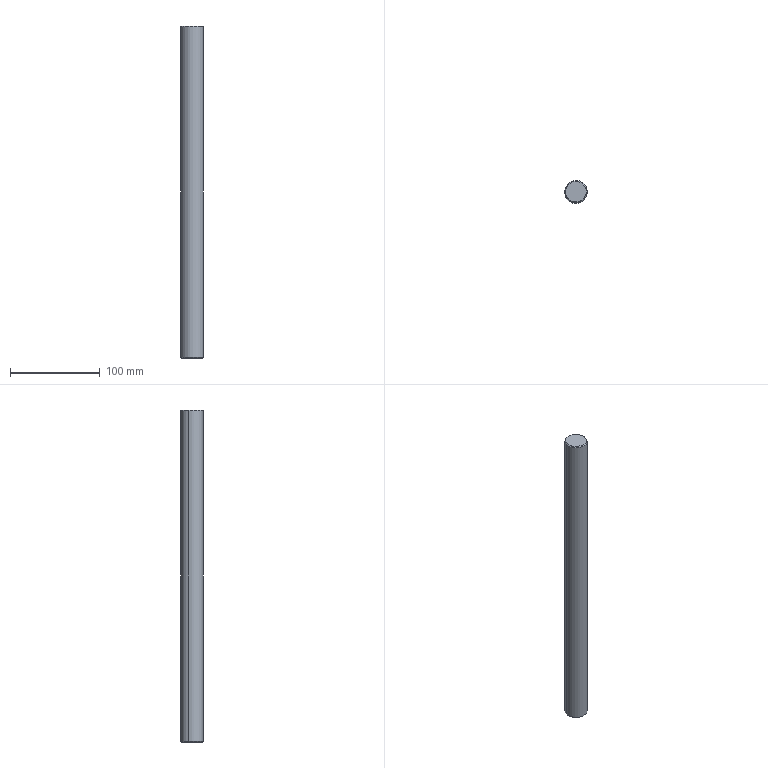Component | SolidWorks | DirectPressureVerticalSeal-1_VerticalSealGuideAxis-2 | 1 solid | 8 faces | box 25 x 25 x 370 mm | volume 181547 mm3 | cone 4 | cylinder 2 | plane 2 | commonest cylinder face diameters 25 x2
build123d program:
from build123d import *


with BuildPart() as part:
    # Sketch1 → Revolve1 (revolve)
    with BuildSketch(Plane.XZ, mode=Mode.PRIVATE) as revolve1_sk:
        Polygon((11.5, 185), (0, 185), (0, -185), (11.5, -185), (12.5, -184), (12.5, 184), align=None)
    revolve(revolve1_sk.sketch.rotate(Axis((0, 0, 185), (0, 0, -1)), 180), axis=Axis((0, 0, 185), (0, 0, -1)))


solid = part.part

# Placed as in the assembly
solid = solid.moved(Location((-98.746, 246.873, 168.5), (0, 0, 0)))
STEP:
#1=COLOUR_RGB('',0.7922,0.8196,0.9333);
#2=FILL_AREA_STYLE_COLOUR('',#1);
#3=FILL_AREA_STYLE('',(#2));
#4=SURFACE_STYLE_FILL_AREA(#3);
#5=SURFACE_SIDE_STYLE('',(#4));
#6=SURFACE_STYLE_USAGE(.BOTH.,#5);
#7=PRESENTATION_STYLE_ASSIGNMENT((#6));
#8=CARTESIAN_POINT('',(-4.323,9.842,-0.6496));
#9=VERTEX_POINT('',#8);
#10=CARTESIAN_POINT('',(-3.452,9.597,-0.6496));
#11=VERTEX_POINT('',#10);
#12=CARTESIAN_POINT('',(-3.888,9.719,-0.6496));
#13=DIRECTION('',(0.,0.,-1.));
#14=DIRECTION('',(-0.9626,0.2708,0.));
#15=AXIS2_PLACEMENT_3D('',#12,#13,#14);
#16=CIRCLE('',#15,0.4528);
#17=EDGE_CURVE('',#9,#11,#16,.T.);
#18=ORIENTED_EDGE('',*,*,#17,.F.);
#19=CARTESIAN_POINT('',(-4.361,9.853,-0.6102));
#20=VERTEX_POINT('',#19);
#21=CARTESIAN_POINT('',(-4.323,9.842,-0.6496));
#22=DIRECTION('',(-0.6807,0.1915,0.7071));
#23=VECTOR('',#22,39.37);
#24=LINE('',#21,#23);
#25=EDGE_CURVE('',#9,#20,#24,.T.);
#26=ORIENTED_EDGE('',*,*,#25,.T.);
#27=CARTESIAN_POINT('',(-3.414,9.586,-0.6102));
#28=VERTEX_POINT('',#27);
#29=CARTESIAN_POINT('',(-3.888,9.719,-0.6102));
#30=DIRECTION('',(0.,0.,-1.));
#31=DIRECTION('',(-0.9626,0.2708,-0.));
#32=AXIS2_PLACEMENT_3D('',#29,#30,#31);
#33=CIRCLE('',#32,0.4921);
#34=EDGE_CURVE('',#20,#28,#33,.T.);
#35=ORIENTED_EDGE('',*,*,#34,.T.);
#36=CARTESIAN_POINT('',(-3.452,9.597,-0.6496));
#37=DIRECTION('',(0.6807,-0.1915,0.7071));
#38=VECTOR('',#37,39.37);
#39=LINE('',#36,#38);
#40=EDGE_CURVE('',#11,#28,#39,.T.);
#41=ORIENTED_EDGE('',*,*,#40,.F.);
#42=EDGE_LOOP('',(#18,#26,#35,#41));
#43=FACE_OUTER_BOUND('',#42,.T.);
#44=CARTESIAN_POINT('',(-3.888,9.719,-0.6496));
#45=DIRECTION('',(-0.,-0.,1.));
#46=DIRECTION('',(0.9626,-0.2708,0.));
#47=AXIS2_PLACEMENT_3D('',#44,#45,#46);
#48=CONICAL_SURFACE('',#47,0.4528,0.7854);
#49=ADVANCED_FACE('',(#43),#48,.T.);
#50=CARTESIAN_POINT('',(-4.361,9.853,13.878));
#51=VERTEX_POINT('',#50);
#52=CARTESIAN_POINT('',(-3.414,9.586,13.878));
#53=VERTEX_POINT('',#52);
#54=CARTESIAN_POINT('',(-3.888,9.719,13.878));
#55=DIRECTION('',(0.,0.,-1.));
#56=DIRECTION('',(-0.9626,0.2708,0.));
#57=AXIS2_PLACEMENT_3D('',#54,#55,#56);
#58=CIRCLE('',#57,0.4921);
#59=EDGE_CURVE('',#51,#53,#58,.T.);
#60=ORIENTED_EDGE('',*,*,#59,.T.);
#61=CARTESIAN_POINT('',(-3.414,9.586,13.917));
#62=DIRECTION('',(0.,0.,-1.));
#63=VECTOR('',#62,39.37);
#64=LINE('',#61,#63);
#65=EDGE_CURVE('',#53,#28,#64,.T.);
#66=ORIENTED_EDGE('',*,*,#65,.T.);
#67=ORIENTED_EDGE('',*,*,#34,.F.);
#68=CARTESIAN_POINT('',(-4.361,9.853,13.917));
#69=DIRECTION('',(0.,0.,-1.));
#70=VECTOR('',#69,39.37);
#71=LINE('',#68,#70);
#72=EDGE_CURVE('',#51,#20,#71,.T.);
#73=ORIENTED_EDGE('',*,*,#72,.F.);
#74=EDGE_LOOP('',(#60,#66,#67,#73));
#75=FACE_OUTER_BOUND('',#74,.T.);
#76=CARTESIAN_POINT('',(-3.888,9.719,13.917));
#77=DIRECTION('',(0.,0.,-1.));
#78=DIRECTION('',(-0.9626,0.2708,0.));
#79=AXIS2_PLACEMENT_3D('',#76,#77,#78);
#80=CYLINDRICAL_SURFACE('',#79,0.4921);
#81=ADVANCED_FACE('',(#75),#80,.T.);
#82=CARTESIAN_POINT('',(-4.323,9.842,13.917));
#83=VERTEX_POINT('',#82);
#84=CARTESIAN_POINT('',(-3.452,9.597,13.917));
#85=VERTEX_POINT('',#84);
#86=CARTESIAN_POINT('',(-3.888,9.719,13.917));
#87=DIRECTION('',(0.,0.,-1.));
#88=DIRECTION('',(-0.9626,0.2708,0.));
#89=AXIS2_PLACEMENT_3D('',#86,#87,#88);
#90=CIRCLE('',#89,0.4528);
#91=EDGE_CURVE('',#83,#85,#90,.T.);
#92=ORIENTED_EDGE('',*,*,#91,.T.);
#93=CARTESIAN_POINT('',(-3.414,9.586,13.878));
#94=DIRECTION('',(0.6807,-0.1915,-0.7071));
#95=VECTOR('',#94,39.37);
#96=LINE('',#93,#95);
#97=EDGE_CURVE('',#85,#53,#96,.T.);
#98=ORIENTED_EDGE('',*,*,#97,.T.);
#99=ORIENTED_EDGE('',*,*,#59,.F.);
#100=CARTESIAN_POINT('',(-4.361,9.853,13.878));
#101=DIRECTION('',(-0.6807,0.1915,-0.7071));
#102=VECTOR('',#101,39.37);
#103=LINE('',#100,#102);
#104=EDGE_CURVE('',#83,#51,#103,.T.);
#105=ORIENTED_EDGE('',*,*,#104,.F.);
#106=EDGE_LOOP('',(#92,#98,#99,#105));
#107=FACE_OUTER_BOUND('',#106,.T.);
#108=CARTESIAN_POINT('',(-3.888,9.719,13.878));
#109=DIRECTION('',(0.,0.,-1.));
#110=DIRECTION('',(-0.9626,0.2708,0.));
#111=AXIS2_PLACEMENT_3D('',#108,#109,#110);
#112=CONICAL_SURFACE('',#111,0.4921,0.7854);
#113=ADVANCED_FACE('',(#107),#112,.T.);
#114=ORIENTED_EDGE('',*,*,#97,.F.);
#115=CARTESIAN_POINT('',(-3.888,9.719,13.917));
#116=DIRECTION('',(0.,0.,-1.));
#117=DIRECTION('',(-0.9626,0.2708,0.));
#118=AXIS2_PLACEMENT_3D('',#115,#116,#117);
#119=CIRCLE('',#118,0.4528);
#120=EDGE_CURVE('',#85,#83,#119,.T.);
#121=ORIENTED_EDGE('',*,*,#120,.T.);
#122=ORIENTED_EDGE('',*,*,#104,.T.);
#123=CARTESIAN_POINT('',(-3.888,9.719,13.878));
#124=DIRECTION('',(0.,0.,-1.));
#125=DIRECTION('',(-0.9626,0.2708,0.));
#126=AXIS2_PLACEMENT_3D('',#123,#124,#125);
#127=CIRCLE('',#126,0.4921);
#128=EDGE_CURVE('',#53,#51,#127,.T.);
#129=ORIENTED_EDGE('',*,*,#128,.F.);
#130=EDGE_LOOP('',(#114,#121,#122,#129));
#131=FACE_OUTER_BOUND('',#130,.T.);
#132=CARTESIAN_POINT('',(-3.888,9.719,13.878));
#133=DIRECTION('',(0.,0.,-1.));
#134=DIRECTION('',(-0.9626,0.2708,0.));
#135=AXIS2_PLACEMENT_3D('',#132,#133,#134);
#136=CONICAL_SURFACE('',#135,0.4921,0.7854);
#137=ADVANCED_FACE('',(#131),#136,.T.);
#138=ORIENTED_EDGE('',*,*,#65,.F.);
#139=ORIENTED_EDGE('',*,*,#128,.T.);
#140=ORIENTED_EDGE('',*,*,#72,.T.);
#141=CARTESIAN_POINT('',(-3.888,9.719,-0.6102));
#142=DIRECTION('',(0.,0.,-1.));
#143=DIRECTION('',(-0.9626,0.2708,-0.));
#144=AXIS2_PLACEMENT_3D('',#141,#142,#143);
#145=CIRCLE('',#144,0.4921);
#146=EDGE_CURVE('',#28,#20,#145,.T.);
#147=ORIENTED_EDGE('',*,*,#146,.F.);
#148=EDGE_LOOP('',(#138,#139,#140,#147));
#149=FACE_OUTER_BOUND('',#148,.T.);
#150=CARTESIAN_POINT('',(-3.888,9.719,13.917));
#151=DIRECTION('',(0.,0.,-1.));
#152=DIRECTION('',(-0.9626,0.2708,0.));
#153=AXIS2_PLACEMENT_3D('',#150,#151,#152);
#154=CYLINDRICAL_SURFACE('',#153,0.4921);
#155=ADVANCED_FACE('',(#149),#154,.T.);
#156=ORIENTED_EDGE('',*,*,#25,.F.);
#157=CARTESIAN_POINT('',(-3.888,9.719,-0.6496));
#158=DIRECTION('',(0.,0.,-1.));
#159=DIRECTION('',(-0.9626,0.2708,0.));
#160=AXIS2_PLACEMENT_3D('',#157,#158,#159);
#161=CIRCLE('',#160,0.4528);
#162=EDGE_CURVE('',#11,#9,#161,.T.);
#163=ORIENTED_EDGE('',*,*,#162,.F.);
#164=ORIENTED_EDGE('',*,*,#40,.T.);
#165=ORIENTED_EDGE('',*,*,#146,.T.);
#166=EDGE_LOOP('',(#156,#163,#164,#165));
#167=FACE_OUTER_BOUND('',#166,.T.);
#168=CARTESIAN_POINT('',(-3.888,9.719,-0.6496));
#169=DIRECTION('',(-0.,-0.,1.));
#170=DIRECTION('',(0.9626,-0.2708,0.));
#171=AXIS2_PLACEMENT_3D('',#168,#169,#170);
#172=CONICAL_SURFACE('',#171,0.4528,0.7854);
#173=ADVANCED_FACE('',(#167),#172,.T.);
#174=ORIENTED_EDGE('',*,*,#162,.T.);
#175=ORIENTED_EDGE('',*,*,#17,.T.);
#176=EDGE_LOOP('',(#174,#175));
#177=FACE_OUTER_BOUND('',#176,.T.);
#178=CARTESIAN_POINT('',(-3.888,9.719,-0.6496));
#179=DIRECTION('',(0.,0.,-1.));
#180=DIRECTION('',(-0.9626,0.2708,-0.));
#181=AXIS2_PLACEMENT_3D('',#178,#179,#180);
#182=PLANE('',#181);
#183=ADVANCED_FACE('',(#177),#182,.T.);
#184=ORIENTED_EDGE('',*,*,#91,.F.);
#185=ORIENTED_EDGE('',*,*,#120,.F.);
#186=EDGE_LOOP('',(#184,#185));
#187=FACE_OUTER_BOUND('',#186,.T.);
#188=CARTESIAN_POINT('',(-3.452,9.597,13.917));
#189=DIRECTION('',(-0.,-0.,1.));
#190=DIRECTION('',(0.9626,-0.2708,0.));
#191=AXIS2_PLACEMENT_3D('',#188,#189,#190);
#192=PLANE('',#191);
#193=ADVANCED_FACE('',(#187),#192,.T.);
#194=CLOSED_SHELL('',(#49,#81,#113,#137,#155,#173,#183,#193));
#195=MANIFOLD_SOLID_BREP('',#194);
#196=STYLED_ITEM('',(#7),#195);
#197=PRESENTATION_LAYER_ASSIGNMENT('','',(#196));
#198=CARTESIAN_POINT('',(0.,0.,0.));
#199=DIRECTION('',(0.,0.,1.));
#200=DIRECTION('',(1.,0.,0.));
#201=AXIS2_PLACEMENT_3D('',#198,#199,#200);
#202=(LENGTH_UNIT()NAMED_UNIT(*)SI_UNIT($,.METRE.));
#203=LENGTH_MEASURE_WITH_UNIT(LENGTH_MEASURE(0.0254),#202);
#204=DIMENSIONAL_EXPONENTS(1.,0.,0.,0.,0.,0.,0.);
#205=(CONVERSION_BASED_UNIT('',#203)LENGTH_UNIT()NAMED_UNIT(#204));
#206=UNCERTAINTY_MEASURE_WITH_UNIT(LENGTH_MEASURE(0.00001),#205,'','');
#207=(NAMED_UNIT(*)PLANE_ANGLE_UNIT()SI_UNIT($,.RADIAN.));
#208=(NAMED_UNIT(*)SI_UNIT($,.STERADIAN.)SOLID_ANGLE_UNIT());
#209=(GEOMETRIC_REPRESENTATION_CONTEXT(3)GLOBAL_UNCERTAINTY_ASSIGNED_CONTEXT((#206))GLOBAL_UNIT_ASSIGNED_CONTEXT((#205,#207,#208))REPRESENTATION_CONTEXT('',''));
#210=ADVANCED_BREP_SHAPE_REPRESENTATION('',(#195,#201),#209);
#211=(LENGTH_UNIT()NAMED_UNIT(*)SI_UNIT($,.METRE.));
#212=LENGTH_MEASURE_WITH_UNIT(LENGTH_MEASURE(0.0254),#211);
#213=DIMENSIONAL_EXPONENTS(1.,0.,0.,0.,0.,0.,0.);
#214=(CONVERSION_BASED_UNIT('',#212)LENGTH_UNIT()NAMED_UNIT(#213));
#215=UNCERTAINTY_MEASURE_WITH_UNIT(LENGTH_MEASURE(0.00001),#214,'','');
#216=(NAMED_UNIT(*)PLANE_ANGLE_UNIT()SI_UNIT($,.RADIAN.));
#217=(NAMED_UNIT(*)SI_UNIT($,.STERADIAN.)SOLID_ANGLE_UNIT());
#218=(GEOMETRIC_REPRESENTATION_CONTEXT(3)GLOBAL_UNCERTAINTY_ASSIGNED_CONTEXT((#215))GLOBAL_UNIT_ASSIGNED_CONTEXT((#214,#216,#217))REPRESENTATION_CONTEXT('',''));
#219=MECHANICAL_DESIGN_GEOMETRIC_PRESENTATION_REPRESENTATION('',(#196),#218);